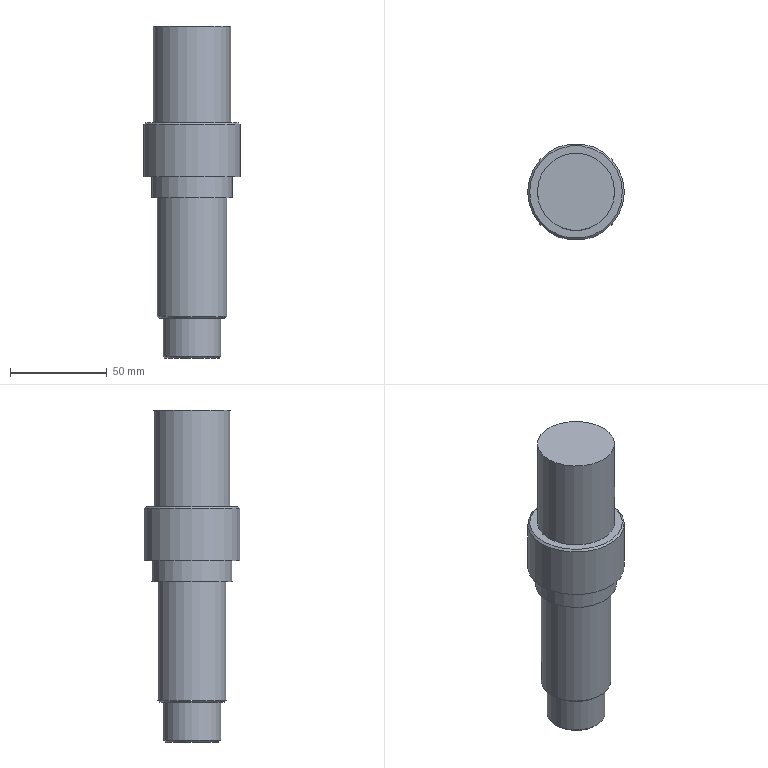Component | NX | SHAFT | 1 solid | 14 faces | box 50 x 50 x 172 mm | volume 210978 mm3 | plane 6 | cylinder 5 | cone 3 | commonest cylinder face diameters 36 x1 42 x1 50 x1 30 x1 40 x1
STEP:
#1=CARTESIAN_POINT('',(0.,0.,0.));
#2=DIRECTION('',(0.,0.,1.));
#3=DIRECTION('',(1.,0.,0.));
#4=AXIS2_PLACEMENT_3D('',#1,#2,#3);
#5=CARTESIAN_POINT('',(109.964,361.403,443.));
#6=VERTEX_POINT('',#5);
#7=CARTESIAN_POINT('',(91.964,361.403,443.));
#8=DIRECTION('',(0.,0.,1.));
#9=DIRECTION('',(1.,0.,0.));
#10=AXIS2_PLACEMENT_3D('',#7,#8,#9);
#11=CIRCLE('',#10,18.);
#12=CARTESIAN_POINT('',(91.964,361.403,543.5));
#13=DIRECTION('',(0.,0.,-1.));
#14=DIRECTION('',(1.,0.,0.));
#15=AXIS2_PLACEMENT_3D('',#12,#13,#14);
#16=CYLINDRICAL_SURFACE('',#15,18.);
#17=CARTESIAN_POINT('',(6.283,100.5));
#18=DIRECTION('',(-1.,0.));
#19=VECTOR('',#18,1.);
#20=LINE('',#17,#19);
#21=(GEOMETRIC_REPRESENTATION_CONTEXT(2)PARAMETRIC_REPRESENTATION_CONTEXT()REPRESENTATION_CONTEXT('',''));
#22=DEFINITIONAL_REPRESENTATION('',(#20),#21);
#23=PCURVE('',#16,#22);
#24=CARTESIAN_POINT('',(91.964,361.403,443.));
#25=DIRECTION('',(0.,0.,1.));
#26=DIRECTION('',(-1.,0.,0.));
#27=AXIS2_PLACEMENT_3D('',#24,#25,#26);
#28=CONICAL_SURFACE('',#27,18.,0.7854);
#29=CARTESIAN_POINT('',(3.142,0.));
#30=DIRECTION('',(1.,0.));
#31=VECTOR('',#30,1.);
#32=LINE('',#29,#31);
#33=(GEOMETRIC_REPRESENTATION_CONTEXT(2)PARAMETRIC_REPRESENTATION_CONTEXT()REPRESENTATION_CONTEXT('',''));
#34=DEFINITIONAL_REPRESENTATION('',(#32),#33);
#35=PCURVE('',#28,#34);
#36=SURFACE_CURVE('',#11,(#23,#35),.PCURVE_S1.);
#37=EDGE_CURVE('',#6,#6,#36,.T.);
#38=ORIENTED_EDGE('',*,*,#37,.T.);
#39=CARTESIAN_POINT('',(109.964,361.403,504.5));
#40=VERTEX_POINT('',#39);
#41=CARTESIAN_POINT('',(109.964,361.403,504.5));
#42=CARTESIAN_POINT('',(109.964,361.403,443.));
#43=B_SPLINE_CURVE_WITH_KNOTS('',1,(#41,#42),.UNSPECIFIED.,.F.,.F.,(2,2),(39.,100.5),.PIECEWISE_BEZIER_KNOTS.);
#44=CARTESIAN_POINT('',(0.,0.));
#45=DIRECTION('',(0.,1.));
#46=VECTOR('',#45,1.);
#47=LINE('',#44,#46);
#48=(GEOMETRIC_REPRESENTATION_CONTEXT(2)PARAMETRIC_REPRESENTATION_CONTEXT()REPRESENTATION_CONTEXT('',''));
#49=DEFINITIONAL_REPRESENTATION('',(#47),#48);
#50=PCURVE('',#16,#49);
#51=CARTESIAN_POINT('',(6.283,0.));
#52=DIRECTION('',(0.,1.));
#53=VECTOR('',#52,1.);
#54=LINE('',#51,#53);
#55=(GEOMETRIC_REPRESENTATION_CONTEXT(2)PARAMETRIC_REPRESENTATION_CONTEXT()REPRESENTATION_CONTEXT('',''));
#56=DEFINITIONAL_REPRESENTATION('',(#54),#55);
#57=PCURVE('',#16,#56);
#58=SEAM_CURVE('',#43,(#50,#57),.PCURVE_S1.);
#59=EDGE_CURVE('',#40,#6,#58,.T.);
#60=ORIENTED_EDGE('',*,*,#59,.F.);
#61=CARTESIAN_POINT('',(91.964,361.403,504.5));
#62=DIRECTION('',(0.,0.,-1.));
#63=DIRECTION('',(1.,0.,0.));
#64=AXIS2_PLACEMENT_3D('',#61,#62,#63);
#65=CIRCLE('',#64,18.);
#66=CARTESIAN_POINT('',(0.,39.));
#67=DIRECTION('',(1.,0.));
#68=VECTOR('',#67,1.);
#69=LINE('',#66,#68);
#70=(GEOMETRIC_REPRESENTATION_CONTEXT(2)PARAMETRIC_REPRESENTATION_CONTEXT()REPRESENTATION_CONTEXT('',''));
#71=DEFINITIONAL_REPRESENTATION('',(#69),#70);
#72=PCURVE('',#16,#71);
#73=CARTESIAN_POINT('',(91.964,361.403,504.5));
#74=DIRECTION('',(0.,0.,-1.));
#75=DIRECTION('',(1.,0.,0.));
#76=AXIS2_PLACEMENT_3D('',#73,#74,#75);
#77=PLANE('',#76);
#78=CARTESIAN_POINT('',(0.,0.));
#79=DIRECTION('',(1.,0.));
#80=AXIS2_PLACEMENT_2D('',#78,#79);
#81=CIRCLE('',#80,18.);
#82=(GEOMETRIC_REPRESENTATION_CONTEXT(2)PARAMETRIC_REPRESENTATION_CONTEXT()REPRESENTATION_CONTEXT('',''));
#83=DEFINITIONAL_REPRESENTATION('',(#81),#82);
#84=PCURVE('',#77,#83);
#85=SURFACE_CURVE('',#65,(#72,#84),.PCURVE_S1.);
#86=EDGE_CURVE('',#40,#40,#85,.T.);
#87=ORIENTED_EDGE('',*,*,#86,.T.);
#88=ORIENTED_EDGE('',*,*,#59,.T.);
#89=EDGE_LOOP('',(#38,#60,#87,#88));
#90=FACE_BOUND('',#89,.T.);
#91=ADVANCED_FACE('',(#90),#16,.T.);
#92=CARTESIAN_POINT('',(112.964,361.403,515.5));
#93=VERTEX_POINT('',#92);
#94=CARTESIAN_POINT('',(91.964,361.403,515.5));
#95=DIRECTION('',(0.,0.,-1.));
#96=DIRECTION('',(1.,0.,0.));
#97=AXIS2_PLACEMENT_3D('',#94,#95,#96);
#98=CIRCLE('',#97,21.);
#99=CARTESIAN_POINT('',(91.964,361.403,515.5));
#100=DIRECTION('',(0.,0.,-1.));
#101=DIRECTION('',(1.,0.,0.));
#102=AXIS2_PLACEMENT_3D('',#99,#100,#101);
#103=PLANE('',#102);
#104=CARTESIAN_POINT('',(0.,0.));
#105=DIRECTION('',(1.,0.));
#106=AXIS2_PLACEMENT_2D('',#104,#105);
#107=CIRCLE('',#106,21.);
#108=(GEOMETRIC_REPRESENTATION_CONTEXT(2)PARAMETRIC_REPRESENTATION_CONTEXT()REPRESENTATION_CONTEXT('',''));
#109=DEFINITIONAL_REPRESENTATION('',(#107),#108);
#110=PCURVE('',#103,#109);
#111=CARTESIAN_POINT('',(91.964,361.403,543.5));
#112=DIRECTION('',(0.,0.,-1.));
#113=DIRECTION('',(1.,0.,0.));
#114=AXIS2_PLACEMENT_3D('',#111,#112,#113);
#115=CYLINDRICAL_SURFACE('',#114,21.);
#116=CARTESIAN_POINT('',(0.,28.));
#117=DIRECTION('',(1.,0.));
#118=VECTOR('',#117,1.);
#119=LINE('',#116,#118);
#120=(GEOMETRIC_REPRESENTATION_CONTEXT(2)PARAMETRIC_REPRESENTATION_CONTEXT()REPRESENTATION_CONTEXT('',''));
#121=DEFINITIONAL_REPRESENTATION('',(#119),#120);
#122=PCURVE('',#115,#121);
#123=SURFACE_CURVE('',#98,(#110,#122),.PCURVE_S1.);
#124=EDGE_CURVE('',#93,#93,#123,.T.);
#125=ORIENTED_EDGE('',*,*,#124,.F.);
#126=EDGE_LOOP('',(#125));
#127=FACE_BOUND('',#126,.T.);
#128=CARTESIAN_POINT('',(116.964,361.403,515.5));
#129=VERTEX_POINT('',#128);
#130=CARTESIAN_POINT('',(91.964,361.403,515.5));
#131=DIRECTION('',(0.,0.,-1.));
#132=DIRECTION('',(1.,0.,0.));
#133=AXIS2_PLACEMENT_3D('',#130,#131,#132);
#134=CIRCLE('',#133,25.);
#135=CARTESIAN_POINT('',(0.,0.));
#136=DIRECTION('',(1.,0.));
#137=AXIS2_PLACEMENT_2D('',#135,#136);
#138=CIRCLE('',#137,25.);
#139=(GEOMETRIC_REPRESENTATION_CONTEXT(2)PARAMETRIC_REPRESENTATION_CONTEXT()REPRESENTATION_CONTEXT('',''));
#140=DEFINITIONAL_REPRESENTATION('',(#138),#139);
#141=PCURVE('',#103,#140);
#142=CARTESIAN_POINT('',(91.964,361.403,543.5));
#143=DIRECTION('',(0.,0.,-1.));
#144=DIRECTION('',(1.,0.,0.));
#145=AXIS2_PLACEMENT_3D('',#142,#143,#144);
#146=CYLINDRICAL_SURFACE('',#145,25.);
#147=CARTESIAN_POINT('',(0.,28.));
#148=DIRECTION('',(1.,0.));
#149=VECTOR('',#148,1.);
#150=LINE('',#147,#149);
#151=(GEOMETRIC_REPRESENTATION_CONTEXT(2)PARAMETRIC_REPRESENTATION_CONTEXT()REPRESENTATION_CONTEXT('',''));
#152=DEFINITIONAL_REPRESENTATION('',(#150),#151);
#153=PCURVE('',#146,#152);
#154=SURFACE_CURVE('',#134,(#141,#153),.PCURVE_S1.);
#155=EDGE_CURVE('',#129,#129,#154,.T.);
#156=ORIENTED_EDGE('',*,*,#155,.T.);
#157=EDGE_LOOP('',(#156));
#158=FACE_BOUND('',#157,.T.);
#159=ADVANCED_FACE('',(#127,#158),#103,.T.);
#160=CARTESIAN_POINT('',(112.964,361.403,504.5));
#161=VERTEX_POINT('',#160);
#162=CARTESIAN_POINT('',(91.964,361.403,504.5));
#163=DIRECTION('',(0.,0.,1.));
#164=DIRECTION('',(1.,0.,0.));
#165=AXIS2_PLACEMENT_3D('',#162,#163,#164);
#166=CIRCLE('',#165,21.);
#167=CARTESIAN_POINT('',(21.,0.));
#168=CARTESIAN_POINT('',(21.,-36.373));
#169=CARTESIAN_POINT('',(-10.5,-18.187));
#170=CARTESIAN_POINT('',(-42.,-0.));
#171=CARTESIAN_POINT('',(-10.5,18.187));
#172=CARTESIAN_POINT('',(21.,36.373));
#173=CARTESIAN_POINT('',(21.,0.));
#174=(BOUNDED_CURVE()B_SPLINE_CURVE(2,(#167,#168,#169,#170,#171,#172,#173),.UNSPECIFIED.,.T.,.F.)B_SPLINE_CURVE_WITH_KNOTS((1,2,2,2,2,1),(-2.094,0.,2.094,4.189,6.283,8.378),.UNSPECIFIED.)CURVE()GEOMETRIC_REPRESENTATION_ITEM()RATIONAL_B_SPLINE_CURVE((1.,0.5,1.,0.5,1.,0.5,1.))REPRESENTATION_ITEM(''));
#175=(GEOMETRIC_REPRESENTATION_CONTEXT(2)PARAMETRIC_REPRESENTATION_CONTEXT()REPRESENTATION_CONTEXT('',''));
#176=DEFINITIONAL_REPRESENTATION('',(#174),#175);
#177=PCURVE('',#77,#176);
#178=CARTESIAN_POINT('',(6.283,39.));
#179=DIRECTION('',(-1.,0.));
#180=VECTOR('',#179,1.);
#181=LINE('',#178,#180);
#182=(GEOMETRIC_REPRESENTATION_CONTEXT(2)PARAMETRIC_REPRESENTATION_CONTEXT()REPRESENTATION_CONTEXT('',''));
#183=DEFINITIONAL_REPRESENTATION('',(#181),#182);
#184=PCURVE('',#115,#183);
#185=SURFACE_CURVE('',#166,(#177,#184),.PCURVE_S1.);
#186=EDGE_CURVE('',#161,#161,#185,.T.);
#187=ORIENTED_EDGE('',*,*,#186,.F.);
#188=EDGE_LOOP('',(#187));
#189=FACE_BOUND('',#188,.T.);
#190=ORIENTED_EDGE('',*,*,#86,.F.);
#191=EDGE_LOOP('',(#190));
#192=FACE_BOUND('',#191,.T.);
#193=ADVANCED_FACE('',(#189,#192),#77,.T.);
#194=ORIENTED_EDGE('',*,*,#124,.T.);
#195=CARTESIAN_POINT('',(112.964,361.403,515.5));
#196=CARTESIAN_POINT('',(112.964,361.403,504.5));
#197=B_SPLINE_CURVE_WITH_KNOTS('',1,(#195,#196),.UNSPECIFIED.,.F.,.F.,(2,2),(28.,39.),.PIECEWISE_BEZIER_KNOTS.);
#198=CARTESIAN_POINT('',(6.283,0.));
#199=DIRECTION('',(0.,1.));
#200=VECTOR('',#199,1.);
#201=LINE('',#198,#200);
#202=(GEOMETRIC_REPRESENTATION_CONTEXT(2)PARAMETRIC_REPRESENTATION_CONTEXT()REPRESENTATION_CONTEXT('',''));
#203=DEFINITIONAL_REPRESENTATION('',(#201),#202);
#204=PCURVE('',#115,#203);
#205=CARTESIAN_POINT('',(0.,0.));
#206=DIRECTION('',(0.,1.));
#207=VECTOR('',#206,1.);
#208=LINE('',#205,#207);
#209=(GEOMETRIC_REPRESENTATION_CONTEXT(2)PARAMETRIC_REPRESENTATION_CONTEXT()REPRESENTATION_CONTEXT('',''));
#210=DEFINITIONAL_REPRESENTATION('',(#208),#209);
#211=PCURVE('',#115,#210);
#212=SEAM_CURVE('',#197,(#204,#211),.PCURVE_S1.);
#213=EDGE_CURVE('',#93,#161,#212,.T.);
#214=ORIENTED_EDGE('',*,*,#213,.T.);
#215=ORIENTED_EDGE('',*,*,#186,.T.);
#216=ORIENTED_EDGE('',*,*,#213,.F.);
#217=EDGE_LOOP('',(#194,#214,#215,#216));
#218=FACE_BOUND('',#217,.T.);
#219=ADVANCED_FACE('',(#218),#115,.T.);
#220=CARTESIAN_POINT('',(111.964,361.403,543.5));
#221=VERTEX_POINT('',#220);
#222=CARTESIAN_POINT('',(91.964,361.403,543.5));
#223=DIRECTION('',(0.,0.,1.));
#224=DIRECTION('',(1.,0.,0.));
#225=AXIS2_PLACEMENT_3D('',#222,#223,#224);
#226=CIRCLE('',#225,20.);
#227=CARTESIAN_POINT('',(91.964,361.403,543.5));
#228=DIRECTION('',(0.,0.,-1.));
#229=DIRECTION('',(1.,0.,0.));
#230=AXIS2_PLACEMENT_3D('',#227,#228,#229);
#231=PLANE('',#230);
#232=CARTESIAN_POINT('',(20.,0.));
#233=CARTESIAN_POINT('',(20.,-34.641));
#234=CARTESIAN_POINT('',(-10.,-17.321));
#235=CARTESIAN_POINT('',(-40.,-0.));
#236=CARTESIAN_POINT('',(-10.,17.321));
#237=CARTESIAN_POINT('',(20.,34.641));
#238=CARTESIAN_POINT('',(20.,0.));
#239=(BOUNDED_CURVE()B_SPLINE_CURVE(2,(#232,#233,#234,#235,#236,#237,#238),.UNSPECIFIED.,.T.,.F.)B_SPLINE_CURVE_WITH_KNOTS((1,2,2,2,2,1),(-2.094,0.,2.094,4.189,6.283,8.378),.UNSPECIFIED.)CURVE()GEOMETRIC_REPRESENTATION_ITEM()RATIONAL_B_SPLINE_CURVE((1.,0.5,1.,0.5,1.,0.5,1.))REPRESENTATION_ITEM(''));
#240=(GEOMETRIC_REPRESENTATION_CONTEXT(2)PARAMETRIC_REPRESENTATION_CONTEXT()REPRESENTATION_CONTEXT('',''));
#241=DEFINITIONAL_REPRESENTATION('',(#239),#240);
#242=PCURVE('',#231,#241);
#243=CARTESIAN_POINT('',(91.964,361.403,543.5));
#244=DIRECTION('',(0.,0.,1.));
#245=DIRECTION('',(1.,0.,0.));
#246=AXIS2_PLACEMENT_3D('',#243,#244,#245);
#247=CYLINDRICAL_SURFACE('',#246,20.);
#248=CARTESIAN_POINT('',(0.,0.));
#249=DIRECTION('',(1.,0.));
#250=VECTOR('',#249,1.);
#251=LINE('',#248,#250);
#252=(GEOMETRIC_REPRESENTATION_CONTEXT(2)PARAMETRIC_REPRESENTATION_CONTEXT()REPRESENTATION_CONTEXT('',''));
#253=DEFINITIONAL_REPRESENTATION('',(#251),#252);
#254=PCURVE('',#247,#253);
#255=SURFACE_CURVE('',#226,(#242,#254),.PCURVE_S1.);
#256=EDGE_CURVE('',#221,#221,#255,.T.);
#257=ORIENTED_EDGE('',*,*,#256,.F.);
#258=EDGE_LOOP('',(#257));
#259=FACE_BOUND('',#258,.T.);
#260=CARTESIAN_POINT('',(115.964,361.403,543.5));
#261=VERTEX_POINT('',#260);
#262=CARTESIAN_POINT('',(91.964,361.403,543.5));
#263=DIRECTION('',(0.,0.,1.));
#264=DIRECTION('',(1.,0.,0.));
#265=AXIS2_PLACEMENT_3D('',#262,#263,#264);
#266=CIRCLE('',#265,24.);
#267=CARTESIAN_POINT('',(24.,0.));
#268=CARTESIAN_POINT('',(24.,-41.569));
#269=CARTESIAN_POINT('',(-12.,-20.785));
#270=CARTESIAN_POINT('',(-48.,-0.));
#271=CARTESIAN_POINT('',(-12.,20.785));
#272=CARTESIAN_POINT('',(24.,41.569));
#273=CARTESIAN_POINT('',(24.,0.));
#274=(BOUNDED_CURVE()B_SPLINE_CURVE(2,(#267,#268,#269,#270,#271,#272,#273),.UNSPECIFIED.,.T.,.F.)B_SPLINE_CURVE_WITH_KNOTS((1,2,2,2,2,1),(-2.094,0.,2.094,4.189,6.283,8.378),.UNSPECIFIED.)CURVE()GEOMETRIC_REPRESENTATION_ITEM()RATIONAL_B_SPLINE_CURVE((1.,0.5,1.,0.5,1.,0.5,1.))REPRESENTATION_ITEM(''));
#275=(GEOMETRIC_REPRESENTATION_CONTEXT(2)PARAMETRIC_REPRESENTATION_CONTEXT()REPRESENTATION_CONTEXT('',''));
#276=DEFINITIONAL_REPRESENTATION('',(#274),#275);
#277=PCURVE('',#231,#276);
#278=CARTESIAN_POINT('',(91.964,361.403,542.5));
#279=DIRECTION('',(0.,0.,-1.));
#280=DIRECTION('',(1.,0.,0.));
#281=AXIS2_PLACEMENT_3D('',#278,#279,#280);
#282=CONICAL_SURFACE('',#281,25.,0.7854);
#283=CARTESIAN_POINT('',(6.283,-1.));
#284=DIRECTION('',(-1.,0.));
#285=VECTOR('',#284,1.);
#286=LINE('',#283,#285);
#287=(GEOMETRIC_REPRESENTATION_CONTEXT(2)PARAMETRIC_REPRESENTATION_CONTEXT()REPRESENTATION_CONTEXT('',''));
#288=DEFINITIONAL_REPRESENTATION('',(#286),#287);
#289=PCURVE('',#282,#288);
#290=SURFACE_CURVE('',#266,(#277,#289),.PCURVE_S1.);
#291=EDGE_CURVE('',#261,#261,#290,.T.);
#292=ORIENTED_EDGE('',*,*,#291,.T.);
#293=EDGE_LOOP('',(#292));
#294=FACE_BOUND('',#293,.T.);
#295=ADVANCED_FACE('',(#259,#294),#231,.F.);
#296=CARTESIAN_POINT('',(116.964,361.403,542.5));
#297=VERTEX_POINT('',#296);
#298=CARTESIAN_POINT('',(91.964,361.403,542.5));
#299=DIRECTION('',(0.,0.,-1.));
#300=DIRECTION('',(1.,0.,0.));
#301=AXIS2_PLACEMENT_3D('',#298,#299,#300);
#302=CIRCLE('',#301,25.);
#303=CARTESIAN_POINT('',(0.,1.));
#304=DIRECTION('',(1.,0.));
#305=VECTOR('',#304,1.);
#306=LINE('',#303,#305);
#307=(GEOMETRIC_REPRESENTATION_CONTEXT(2)PARAMETRIC_REPRESENTATION_CONTEXT()REPRESENTATION_CONTEXT('',''));
#308=DEFINITIONAL_REPRESENTATION('',(#306),#307);
#309=PCURVE('',#146,#308);
#310=CARTESIAN_POINT('',(0.,0.));
#311=DIRECTION('',(1.,0.));
#312=VECTOR('',#311,1.);
#313=LINE('',#310,#312);
#314=(GEOMETRIC_REPRESENTATION_CONTEXT(2)PARAMETRIC_REPRESENTATION_CONTEXT()REPRESENTATION_CONTEXT('',''));
#315=DEFINITIONAL_REPRESENTATION('',(#313),#314);
#316=PCURVE('',#282,#315);
#317=SURFACE_CURVE('',#302,(#309,#316),.PCURVE_S1.);
#318=EDGE_CURVE('',#297,#297,#317,.T.);
#319=ORIENTED_EDGE('',*,*,#318,.T.);
#320=CARTESIAN_POINT('',(116.964,361.403,542.5));
#321=CARTESIAN_POINT('',(116.964,361.403,515.5));
#322=B_SPLINE_CURVE_WITH_KNOTS('',1,(#320,#321),.UNSPECIFIED.,.F.,.F.,(2,2),(1.,28.),.PIECEWISE_BEZIER_KNOTS.);
#323=CARTESIAN_POINT('',(6.283,0.));
#324=DIRECTION('',(0.,1.));
#325=VECTOR('',#324,1.);
#326=LINE('',#323,#325);
#327=(GEOMETRIC_REPRESENTATION_CONTEXT(2)PARAMETRIC_REPRESENTATION_CONTEXT()REPRESENTATION_CONTEXT('',''));
#328=DEFINITIONAL_REPRESENTATION('',(#326),#327);
#329=PCURVE('',#146,#328);
#330=CARTESIAN_POINT('',(0.,0.));
#331=DIRECTION('',(0.,1.));
#332=VECTOR('',#331,1.);
#333=LINE('',#330,#332);
#334=(GEOMETRIC_REPRESENTATION_CONTEXT(2)PARAMETRIC_REPRESENTATION_CONTEXT()REPRESENTATION_CONTEXT('',''));
#335=DEFINITIONAL_REPRESENTATION('',(#333),#334);
#336=PCURVE('',#146,#335);
#337=SEAM_CURVE('',#322,(#329,#336),.PCURVE_S1.);
#338=EDGE_CURVE('',#297,#129,#337,.T.);
#339=ORIENTED_EDGE('',*,*,#338,.T.);
#340=ORIENTED_EDGE('',*,*,#155,.F.);
#341=ORIENTED_EDGE('',*,*,#338,.F.);
#342=EDGE_LOOP('',(#319,#339,#340,#341));
#343=FACE_BOUND('',#342,.T.);
#344=ADVANCED_FACE('',(#343),#146,.T.);
#345=CARTESIAN_POINT('',(106.964,361.403,422.5));
#346=VERTEX_POINT('',#345);
#347=CARTESIAN_POINT('',(91.964,361.403,422.5));
#348=DIRECTION('',(0.,0.,1.));
#349=DIRECTION('',(1.,0.,0.));
#350=AXIS2_PLACEMENT_3D('',#347,#348,#349);
#351=CIRCLE('',#350,15.);
#352=CARTESIAN_POINT('',(91.964,361.403,442.));
#353=DIRECTION('',(0.,0.,-1.));
#354=DIRECTION('',(1.,0.,0.));
#355=AXIS2_PLACEMENT_3D('',#352,#353,#354);
#356=CYLINDRICAL_SURFACE('',#355,15.);
#357=CARTESIAN_POINT('',(6.283,19.5));
#358=DIRECTION('',(-1.,0.));
#359=VECTOR('',#358,1.);
#360=LINE('',#357,#359);
#361=(GEOMETRIC_REPRESENTATION_CONTEXT(2)PARAMETRIC_REPRESENTATION_CONTEXT()REPRESENTATION_CONTEXT('',''));
#362=DEFINITIONAL_REPRESENTATION('',(#360),#361);
#363=PCURVE('',#356,#362);
#364=CARTESIAN_POINT('',(91.964,361.403,421.5));
#365=DIRECTION('',(0.,0.,1.));
#366=DIRECTION('',(-1.,0.,0.));
#367=AXIS2_PLACEMENT_3D('',#364,#365,#366);
#368=CONICAL_SURFACE('',#367,14.,0.7854);
#369=CARTESIAN_POINT('',(3.142,1.));
#370=DIRECTION('',(1.,0.));
#371=VECTOR('',#370,1.);
#372=LINE('',#369,#371);
#373=(GEOMETRIC_REPRESENTATION_CONTEXT(2)PARAMETRIC_REPRESENTATION_CONTEXT()REPRESENTATION_CONTEXT('',''));
#374=DEFINITIONAL_REPRESENTATION('',(#372),#373);
#375=PCURVE('',#368,#374);
#376=SURFACE_CURVE('',#351,(#363,#375),.PCURVE_S1.);
#377=EDGE_CURVE('',#346,#346,#376,.T.);
#378=ORIENTED_EDGE('',*,*,#377,.T.);
#379=CARTESIAN_POINT('',(106.964,361.403,442.));
#380=VERTEX_POINT('',#379);
#381=CARTESIAN_POINT('',(106.964,361.403,442.));
#382=CARTESIAN_POINT('',(106.964,361.403,422.5));
#383=B_SPLINE_CURVE_WITH_KNOTS('',1,(#381,#382),.UNSPECIFIED.,.F.,.F.,(2,2),(0.,19.5),.PIECEWISE_BEZIER_KNOTS.);
#384=CARTESIAN_POINT('',(0.,0.));
#385=DIRECTION('',(0.,1.));
#386=VECTOR('',#385,1.);
#387=LINE('',#384,#386);
#388=(GEOMETRIC_REPRESENTATION_CONTEXT(2)PARAMETRIC_REPRESENTATION_CONTEXT()REPRESENTATION_CONTEXT('',''));
#389=DEFINITIONAL_REPRESENTATION('',(#387),#388);
#390=PCURVE('',#356,#389);
#391=CARTESIAN_POINT('',(6.283,0.));
#392=DIRECTION('',(0.,1.));
#393=VECTOR('',#392,1.);
#394=LINE('',#391,#393);
#395=(GEOMETRIC_REPRESENTATION_CONTEXT(2)PARAMETRIC_REPRESENTATION_CONTEXT()REPRESENTATION_CONTEXT('',''));
#396=DEFINITIONAL_REPRESENTATION('',(#394),#395);
#397=PCURVE('',#356,#396);
#398=SEAM_CURVE('',#383,(#390,#397),.PCURVE_S1.);
#399=EDGE_CURVE('',#380,#346,#398,.T.);
#400=ORIENTED_EDGE('',*,*,#399,.F.);
#401=CARTESIAN_POINT('',(91.964,361.403,442.));
#402=DIRECTION('',(0.,0.,1.));
#403=DIRECTION('',(1.,0.,0.));
#404=AXIS2_PLACEMENT_3D('',#401,#402,#403);
#405=CIRCLE('',#404,15.);
#406=CARTESIAN_POINT('',(6.283,0.));
#407=DIRECTION('',(-1.,0.));
#408=VECTOR('',#407,1.);
#409=LINE('',#406,#408);
#410=(GEOMETRIC_REPRESENTATION_CONTEXT(2)PARAMETRIC_REPRESENTATION_CONTEXT()REPRESENTATION_CONTEXT('',''));
#411=DEFINITIONAL_REPRESENTATION('',(#409),#410);
#412=PCURVE('',#356,#411);
#413=CARTESIAN_POINT('',(91.964,361.403,442.));
#414=DIRECTION('',(0.,0.,-1.));
#415=DIRECTION('',(1.,0.,0.));
#416=AXIS2_PLACEMENT_3D('',#413,#414,#415);
#417=PLANE('',#416);
#418=CARTESIAN_POINT('',(15.,0.));
#419=CARTESIAN_POINT('',(15.,-25.981));
#420=CARTESIAN_POINT('',(-7.5,-12.99));
#421=CARTESIAN_POINT('',(-30.,-0.));
#422=CARTESIAN_POINT('',(-7.5,12.99));
#423=CARTESIAN_POINT('',(15.,25.981));
#424=CARTESIAN_POINT('',(15.,0.));
#425=(BOUNDED_CURVE()B_SPLINE_CURVE(2,(#418,#419,#420,#421,#422,#423,#424),.UNSPECIFIED.,.T.,.F.)B_SPLINE_CURVE_WITH_KNOTS((1,2,2,2,2,1),(-2.094,0.,2.094,4.189,6.283,8.378),.UNSPECIFIED.)CURVE()GEOMETRIC_REPRESENTATION_ITEM()RATIONAL_B_SPLINE_CURVE((1.,0.5,1.,0.5,1.,0.5,1.))REPRESENTATION_ITEM(''));
#426=(GEOMETRIC_REPRESENTATION_CONTEXT(2)PARAMETRIC_REPRESENTATION_CONTEXT()REPRESENTATION_CONTEXT('',''));
#427=DEFINITIONAL_REPRESENTATION('',(#425),#426);
#428=PCURVE('',#417,#427);
#429=SURFACE_CURVE('',#405,(#412,#428),.PCURVE_S1.);
#430=EDGE_CURVE('',#380,#380,#429,.T.);
#431=ORIENTED_EDGE('',*,*,#430,.F.);
#432=ORIENTED_EDGE('',*,*,#399,.T.);
#433=EDGE_LOOP('',(#378,#400,#431,#432));
#434=FACE_BOUND('',#433,.T.);
#435=ADVANCED_FACE('',(#434),#356,.T.);
#436=CARTESIAN_POINT('',(108.964,361.403,442.));
#437=VERTEX_POINT('',#436);
#438=CARTESIAN_POINT('',(91.964,361.403,442.));
#439=DIRECTION('',(0.,0.,-1.));
#440=DIRECTION('',(1.,0.,0.));
#441=AXIS2_PLACEMENT_3D('',#438,#439,#440);
#442=CIRCLE('',#441,17.);
#443=CARTESIAN_POINT('',(0.,0.));
#444=DIRECTION('',(1.,0.));
#445=AXIS2_PLACEMENT_2D('',#443,#444);
#446=CIRCLE('',#445,17.);
#447=(GEOMETRIC_REPRESENTATION_CONTEXT(2)PARAMETRIC_REPRESENTATION_CONTEXT()REPRESENTATION_CONTEXT('',''));
#448=DEFINITIONAL_REPRESENTATION('',(#446),#447);
#449=PCURVE('',#417,#448);
#450=CARTESIAN_POINT('',(9.425,-1.));
#451=DIRECTION('',(-1.,0.));
#452=VECTOR('',#451,1.);
#453=LINE('',#450,#452);
#454=(GEOMETRIC_REPRESENTATION_CONTEXT(2)PARAMETRIC_REPRESENTATION_CONTEXT()REPRESENTATION_CONTEXT('',''));
#455=DEFINITIONAL_REPRESENTATION('',(#453),#454);
#456=PCURVE('',#28,#455);
#457=SURFACE_CURVE('',#442,(#449,#456),.PCURVE_S1.);
#458=EDGE_CURVE('',#437,#437,#457,.T.);
#459=ORIENTED_EDGE('',*,*,#458,.T.);
#460=EDGE_LOOP('',(#459));
#461=FACE_BOUND('',#460,.T.);
#462=ORIENTED_EDGE('',*,*,#430,.T.);
#463=EDGE_LOOP('',(#462));
#464=FACE_BOUND('',#463,.T.);
#465=ADVANCED_FACE('',(#461,#464),#417,.T.);
#466=CARTESIAN_POINT('',(105.964,361.403,421.5));
#467=VERTEX_POINT('',#466);
#468=CARTESIAN_POINT('',(91.964,361.403,421.5));
#469=DIRECTION('',(0.,0.,-1.));
#470=DIRECTION('',(1.,0.,0.));
#471=AXIS2_PLACEMENT_3D('',#468,#469,#470);
#472=CIRCLE('',#471,14.);
#473=CARTESIAN_POINT('',(91.964,361.403,421.5));
#474=DIRECTION('',(0.,0.,-1.));
#475=DIRECTION('',(1.,0.,0.));
#476=AXIS2_PLACEMENT_3D('',#473,#474,#475);
#477=PLANE('',#476);
#478=CARTESIAN_POINT('',(0.,0.));
#479=DIRECTION('',(1.,0.));
#480=AXIS2_PLACEMENT_2D('',#478,#479);
#481=CIRCLE('',#480,14.);
#482=(GEOMETRIC_REPRESENTATION_CONTEXT(2)PARAMETRIC_REPRESENTATION_CONTEXT()REPRESENTATION_CONTEXT('',''));
#483=DEFINITIONAL_REPRESENTATION('',(#481),#482);
#484=PCURVE('',#477,#483);
#485=CARTESIAN_POINT('',(9.425,0.));
#486=DIRECTION('',(-1.,0.));
#487=VECTOR('',#486,1.);
#488=LINE('',#485,#487);
#489=(GEOMETRIC_REPRESENTATION_CONTEXT(2)PARAMETRIC_REPRESENTATION_CONTEXT()REPRESENTATION_CONTEXT('',''));
#490=DEFINITIONAL_REPRESENTATION('',(#488),#489);
#491=PCURVE('',#368,#490);
#492=SURFACE_CURVE('',#472,(#484,#491),.PCURVE_S1.);
#493=EDGE_CURVE('',#467,#467,#492,.T.);
#494=ORIENTED_EDGE('',*,*,#493,.T.);
#495=EDGE_LOOP('',(#494));
#496=FACE_BOUND('',#495,.T.);
#497=ADVANCED_FACE('',(#496),#477,.T.);
#498=ORIENTED_EDGE('',*,*,#377,.F.);
#499=CARTESIAN_POINT('',(105.964,361.403,421.5));
#500=CARTESIAN_POINT('',(106.964,361.403,422.5));
#501=B_SPLINE_CURVE_WITH_KNOTS('',1,(#499,#500),.UNSPECIFIED.,.F.,.F.,(2,2),(0.,1.414),.PIECEWISE_BEZIER_KNOTS.);
#502=CARTESIAN_POINT('',(3.142,0.));
#503=DIRECTION('',(0.,1.));
#504=VECTOR('',#503,1.);
#505=LINE('',#502,#504);
#506=(GEOMETRIC_REPRESENTATION_CONTEXT(2)PARAMETRIC_REPRESENTATION_CONTEXT()REPRESENTATION_CONTEXT('',''));
#507=DEFINITIONAL_REPRESENTATION('',(#505),#506);
#508=PCURVE('',#368,#507);
#509=CARTESIAN_POINT('',(9.425,0.));
#510=DIRECTION('',(0.,1.));
#511=VECTOR('',#510,1.);
#512=LINE('',#509,#511);
#513=(GEOMETRIC_REPRESENTATION_CONTEXT(2)PARAMETRIC_REPRESENTATION_CONTEXT()REPRESENTATION_CONTEXT('',''));
#514=DEFINITIONAL_REPRESENTATION('',(#512),#513);
#515=PCURVE('',#368,#514);
#516=SEAM_CURVE('',#501,(#508,#515),.PCURVE_S1.);
#517=EDGE_CURVE('',#467,#346,#516,.T.);
#518=ORIENTED_EDGE('',*,*,#517,.F.);
#519=ORIENTED_EDGE('',*,*,#493,.F.);
#520=ORIENTED_EDGE('',*,*,#517,.T.);
#521=EDGE_LOOP('',(#498,#518,#519,#520));
#522=FACE_BOUND('',#521,.T.);
#523=ADVANCED_FACE('',(#522),#368,.T.);
#524=ORIENTED_EDGE('',*,*,#458,.F.);
#525=CARTESIAN_POINT('',(108.964,361.403,442.));
#526=CARTESIAN_POINT('',(109.964,361.403,443.));
#527=B_SPLINE_CURVE_WITH_KNOTS('',1,(#525,#526),.UNSPECIFIED.,.F.,.F.,(2,2),(-1.414,0.),.PIECEWISE_BEZIER_KNOTS.);
#528=CARTESIAN_POINT('',(9.425,0.));
#529=DIRECTION('',(0.,1.));
#530=VECTOR('',#529,1.);
#531=LINE('',#528,#530);
#532=(GEOMETRIC_REPRESENTATION_CONTEXT(2)PARAMETRIC_REPRESENTATION_CONTEXT()REPRESENTATION_CONTEXT('',''));
#533=DEFINITIONAL_REPRESENTATION('',(#531),#532);
#534=PCURVE('',#28,#533);
#535=CARTESIAN_POINT('',(3.142,0.));
#536=DIRECTION('',(0.,1.));
#537=VECTOR('',#536,1.);
#538=LINE('',#535,#537);
#539=(GEOMETRIC_REPRESENTATION_CONTEXT(2)PARAMETRIC_REPRESENTATION_CONTEXT()REPRESENTATION_CONTEXT('',''));
#540=DEFINITIONAL_REPRESENTATION('',(#538),#539);
#541=PCURVE('',#28,#540);
#542=SEAM_CURVE('',#527,(#534,#541),.PCURVE_S1.);
#543=EDGE_CURVE('',#437,#6,#542,.T.);
#544=ORIENTED_EDGE('',*,*,#543,.T.);
#545=ORIENTED_EDGE('',*,*,#37,.F.);
#546=ORIENTED_EDGE('',*,*,#543,.F.);
#547=EDGE_LOOP('',(#524,#544,#545,#546));
#548=FACE_BOUND('',#547,.T.);
#549=ADVANCED_FACE('',(#548),#28,.T.);
#550=ORIENTED_EDGE('',*,*,#291,.F.);
#551=CARTESIAN_POINT('',(115.964,361.403,543.5));
#552=CARTESIAN_POINT('',(116.964,361.403,542.5));
#553=B_SPLINE_CURVE_WITH_KNOTS('',1,(#551,#552),.UNSPECIFIED.,.F.,.F.,(2,2),(-1.414,0.),.PIECEWISE_BEZIER_KNOTS.);
#554=CARTESIAN_POINT('',(6.283,0.));
#555=DIRECTION('',(0.,1.));
#556=VECTOR('',#555,1.);
#557=LINE('',#554,#556);
#558=(GEOMETRIC_REPRESENTATION_CONTEXT(2)PARAMETRIC_REPRESENTATION_CONTEXT()REPRESENTATION_CONTEXT('',''));
#559=DEFINITIONAL_REPRESENTATION('',(#557),#558);
#560=PCURVE('',#282,#559);
#561=CARTESIAN_POINT('',(0.,0.));
#562=DIRECTION('',(0.,1.));
#563=VECTOR('',#562,1.);
#564=LINE('',#561,#563);
#565=(GEOMETRIC_REPRESENTATION_CONTEXT(2)PARAMETRIC_REPRESENTATION_CONTEXT()REPRESENTATION_CONTEXT('',''));
#566=DEFINITIONAL_REPRESENTATION('',(#564),#565);
#567=PCURVE('',#282,#566);
#568=SEAM_CURVE('',#553,(#560,#567),.PCURVE_S1.);
#569=EDGE_CURVE('',#261,#297,#568,.T.);
#570=ORIENTED_EDGE('',*,*,#569,.T.);
#571=ORIENTED_EDGE('',*,*,#318,.F.);
#572=ORIENTED_EDGE('',*,*,#569,.F.);
#573=EDGE_LOOP('',(#550,#570,#571,#572));
#574=FACE_BOUND('',#573,.T.);
#575=ADVANCED_FACE('',(#574),#282,.T.);
#576=CARTESIAN_POINT('',(111.964,361.403,593.5));
#577=VERTEX_POINT('',#576);
#578=CARTESIAN_POINT('',(91.964,361.403,593.5));
#579=DIRECTION('',(0.,0.,-1.));
#580=DIRECTION('',(1.,0.,0.));
#581=AXIS2_PLACEMENT_3D('',#578,#579,#580);
#582=CIRCLE('',#581,20.);
#583=CARTESIAN_POINT('',(91.964,361.403,593.5));
#584=DIRECTION('',(0.,0.,1.));
#585=DIRECTION('',(-1.,0.,0.));
#586=AXIS2_PLACEMENT_3D('',#583,#584,#585);
#587=PLANE('',#586);
#588=CARTESIAN_POINT('',(-20.,0.));
#589=CARTESIAN_POINT('',(-20.,34.641));
#590=CARTESIAN_POINT('',(10.,17.321));
#591=CARTESIAN_POINT('',(40.,0.));
#592=CARTESIAN_POINT('',(10.,-17.321));
#593=CARTESIAN_POINT('',(-20.,-34.641));
#594=CARTESIAN_POINT('',(-20.,0.));
#595=(BOUNDED_CURVE()B_SPLINE_CURVE(2,(#588,#589,#590,#591,#592,#593,#594),.UNSPECIFIED.,.T.,.F.)B_SPLINE_CURVE_WITH_KNOTS((1,2,2,2,2,1),(-2.094,0.,2.094,4.189,6.283,8.378),.UNSPECIFIED.)CURVE()GEOMETRIC_REPRESENTATION_ITEM()RATIONAL_B_SPLINE_CURVE((1.,0.5,1.,0.5,1.,0.5,1.))REPRESENTATION_ITEM(''));
#596=(GEOMETRIC_REPRESENTATION_CONTEXT(2)PARAMETRIC_REPRESENTATION_CONTEXT()REPRESENTATION_CONTEXT('',''));
#597=DEFINITIONAL_REPRESENTATION('',(#595),#596);
#598=PCURVE('',#587,#597);
#599=CARTESIAN_POINT('',(6.283,50.));
#600=DIRECTION('',(-1.,0.));
#601=VECTOR('',#600,1.);
#602=LINE('',#599,#601);
#603=(GEOMETRIC_REPRESENTATION_CONTEXT(2)PARAMETRIC_REPRESENTATION_CONTEXT()REPRESENTATION_CONTEXT('',''));
#604=DEFINITIONAL_REPRESENTATION('',(#602),#603);
#605=PCURVE('',#247,#604);
#606=SURFACE_CURVE('',#582,(#598,#605),.PCURVE_S1.);
#607=EDGE_CURVE('',#577,#577,#606,.T.);
#608=ORIENTED_EDGE('',*,*,#607,.F.);
#609=EDGE_LOOP('',(#608));
#610=FACE_BOUND('',#609,.T.);
#611=ADVANCED_FACE('',(#610),#587,.T.);
#612=ORIENTED_EDGE('',*,*,#607,.T.);
#613=CARTESIAN_POINT('',(111.964,361.403,543.5));
#614=CARTESIAN_POINT('',(111.964,361.403,593.5));
#615=B_SPLINE_CURVE_WITH_KNOTS('',1,(#613,#614),.UNSPECIFIED.,.F.,.F.,(2,2),(0.,50.),.PIECEWISE_BEZIER_KNOTS.);
#616=CARTESIAN_POINT('',(0.,0.));
#617=DIRECTION('',(0.,1.));
#618=VECTOR('',#617,1.);
#619=LINE('',#616,#618);
#620=(GEOMETRIC_REPRESENTATION_CONTEXT(2)PARAMETRIC_REPRESENTATION_CONTEXT()REPRESENTATION_CONTEXT('',''));
#621=DEFINITIONAL_REPRESENTATION('',(#619),#620);
#622=PCURVE('',#247,#621);
#623=CARTESIAN_POINT('',(6.283,0.));
#624=DIRECTION('',(0.,1.));
#625=VECTOR('',#624,1.);
#626=LINE('',#623,#625);
#627=(GEOMETRIC_REPRESENTATION_CONTEXT(2)PARAMETRIC_REPRESENTATION_CONTEXT()REPRESENTATION_CONTEXT('',''));
#628=DEFINITIONAL_REPRESENTATION('',(#626),#627);
#629=PCURVE('',#247,#628);
#630=SEAM_CURVE('',#615,(#622,#629),.PCURVE_S1.);
#631=EDGE_CURVE('',#221,#577,#630,.T.);
#632=ORIENTED_EDGE('',*,*,#631,.F.);
#633=ORIENTED_EDGE('',*,*,#256,.T.);
#634=ORIENTED_EDGE('',*,*,#631,.T.);
#635=EDGE_LOOP('',(#612,#632,#633,#634));
#636=FACE_BOUND('',#635,.T.);
#637=ADVANCED_FACE('',(#636),#247,.T.);
#638=CLOSED_SHELL('',(#91,#159,#193,#219,#295,#344,#435,#465,#497,#523,#549,#575,#611,#637));
#639=MANIFOLD_SOLID_BREP('',#638);
#640=(LENGTH_UNIT()NAMED_UNIT(*)SI_UNIT(.MILLI.,.METRE.));
#641=UNCERTAINTY_MEASURE_WITH_UNIT(LENGTH_MEASURE(0.00001),#640,'','');
#642=(NAMED_UNIT(*)PLANE_ANGLE_UNIT()SI_UNIT($,.RADIAN.));
#643=(NAMED_UNIT(*)SI_UNIT($,.STERADIAN.)SOLID_ANGLE_UNIT());
#644=(GEOMETRIC_REPRESENTATION_CONTEXT(3)GLOBAL_UNCERTAINTY_ASSIGNED_CONTEXT((#641))GLOBAL_UNIT_ASSIGNED_CONTEXT((#640,#642,#643))REPRESENTATION_CONTEXT('',''));
#645=ADVANCED_BREP_SHAPE_REPRESENTATION('',(#4,#639),#644);